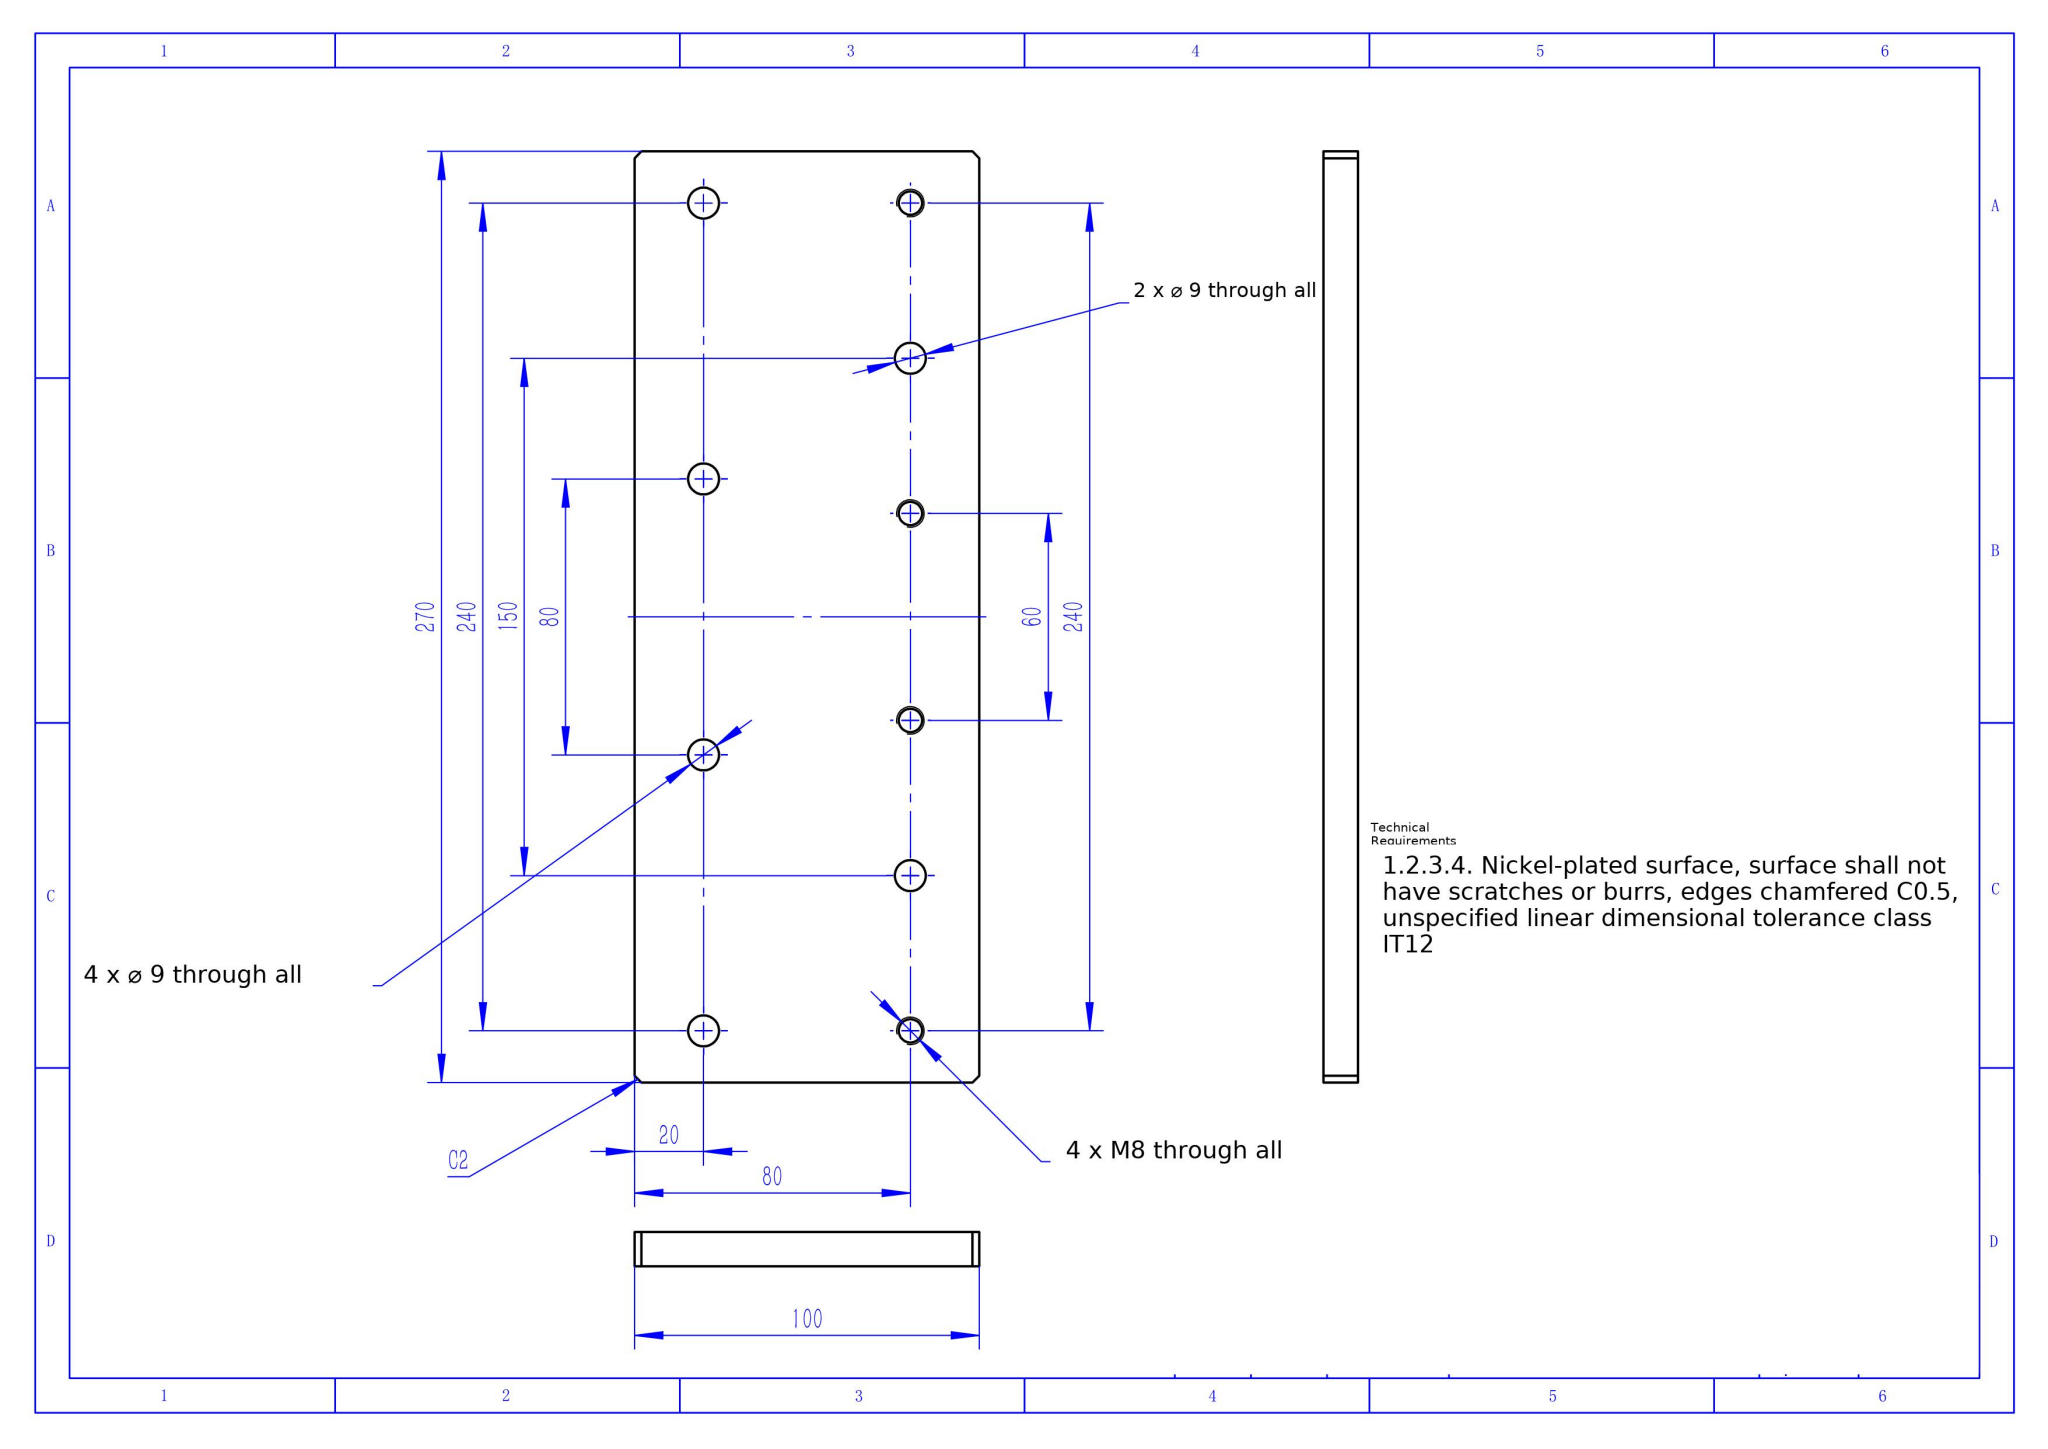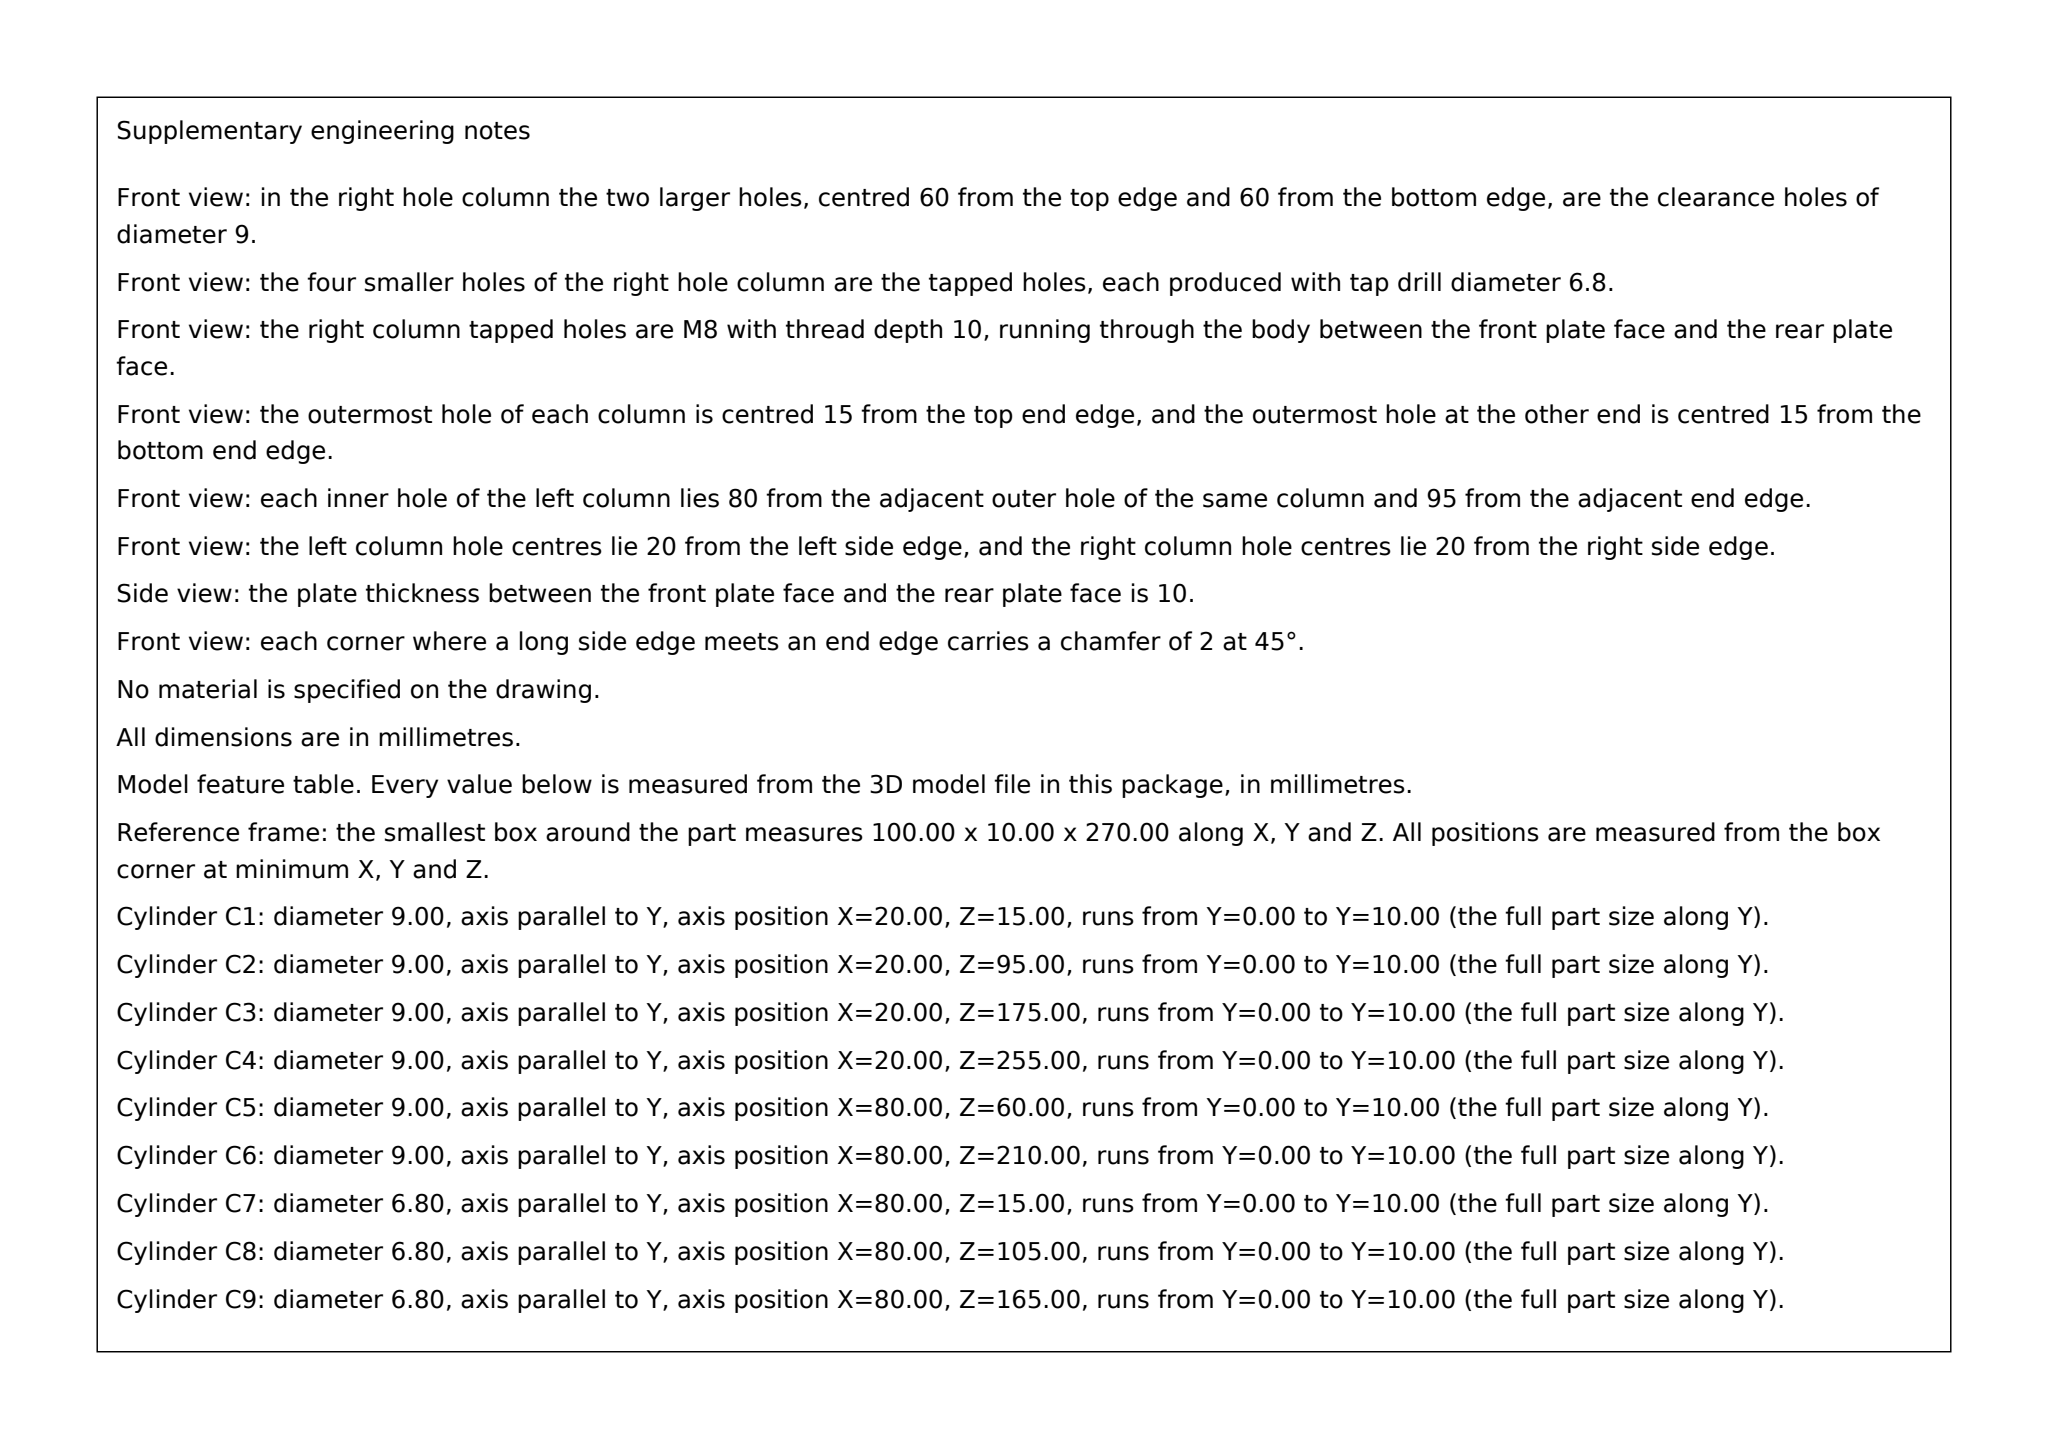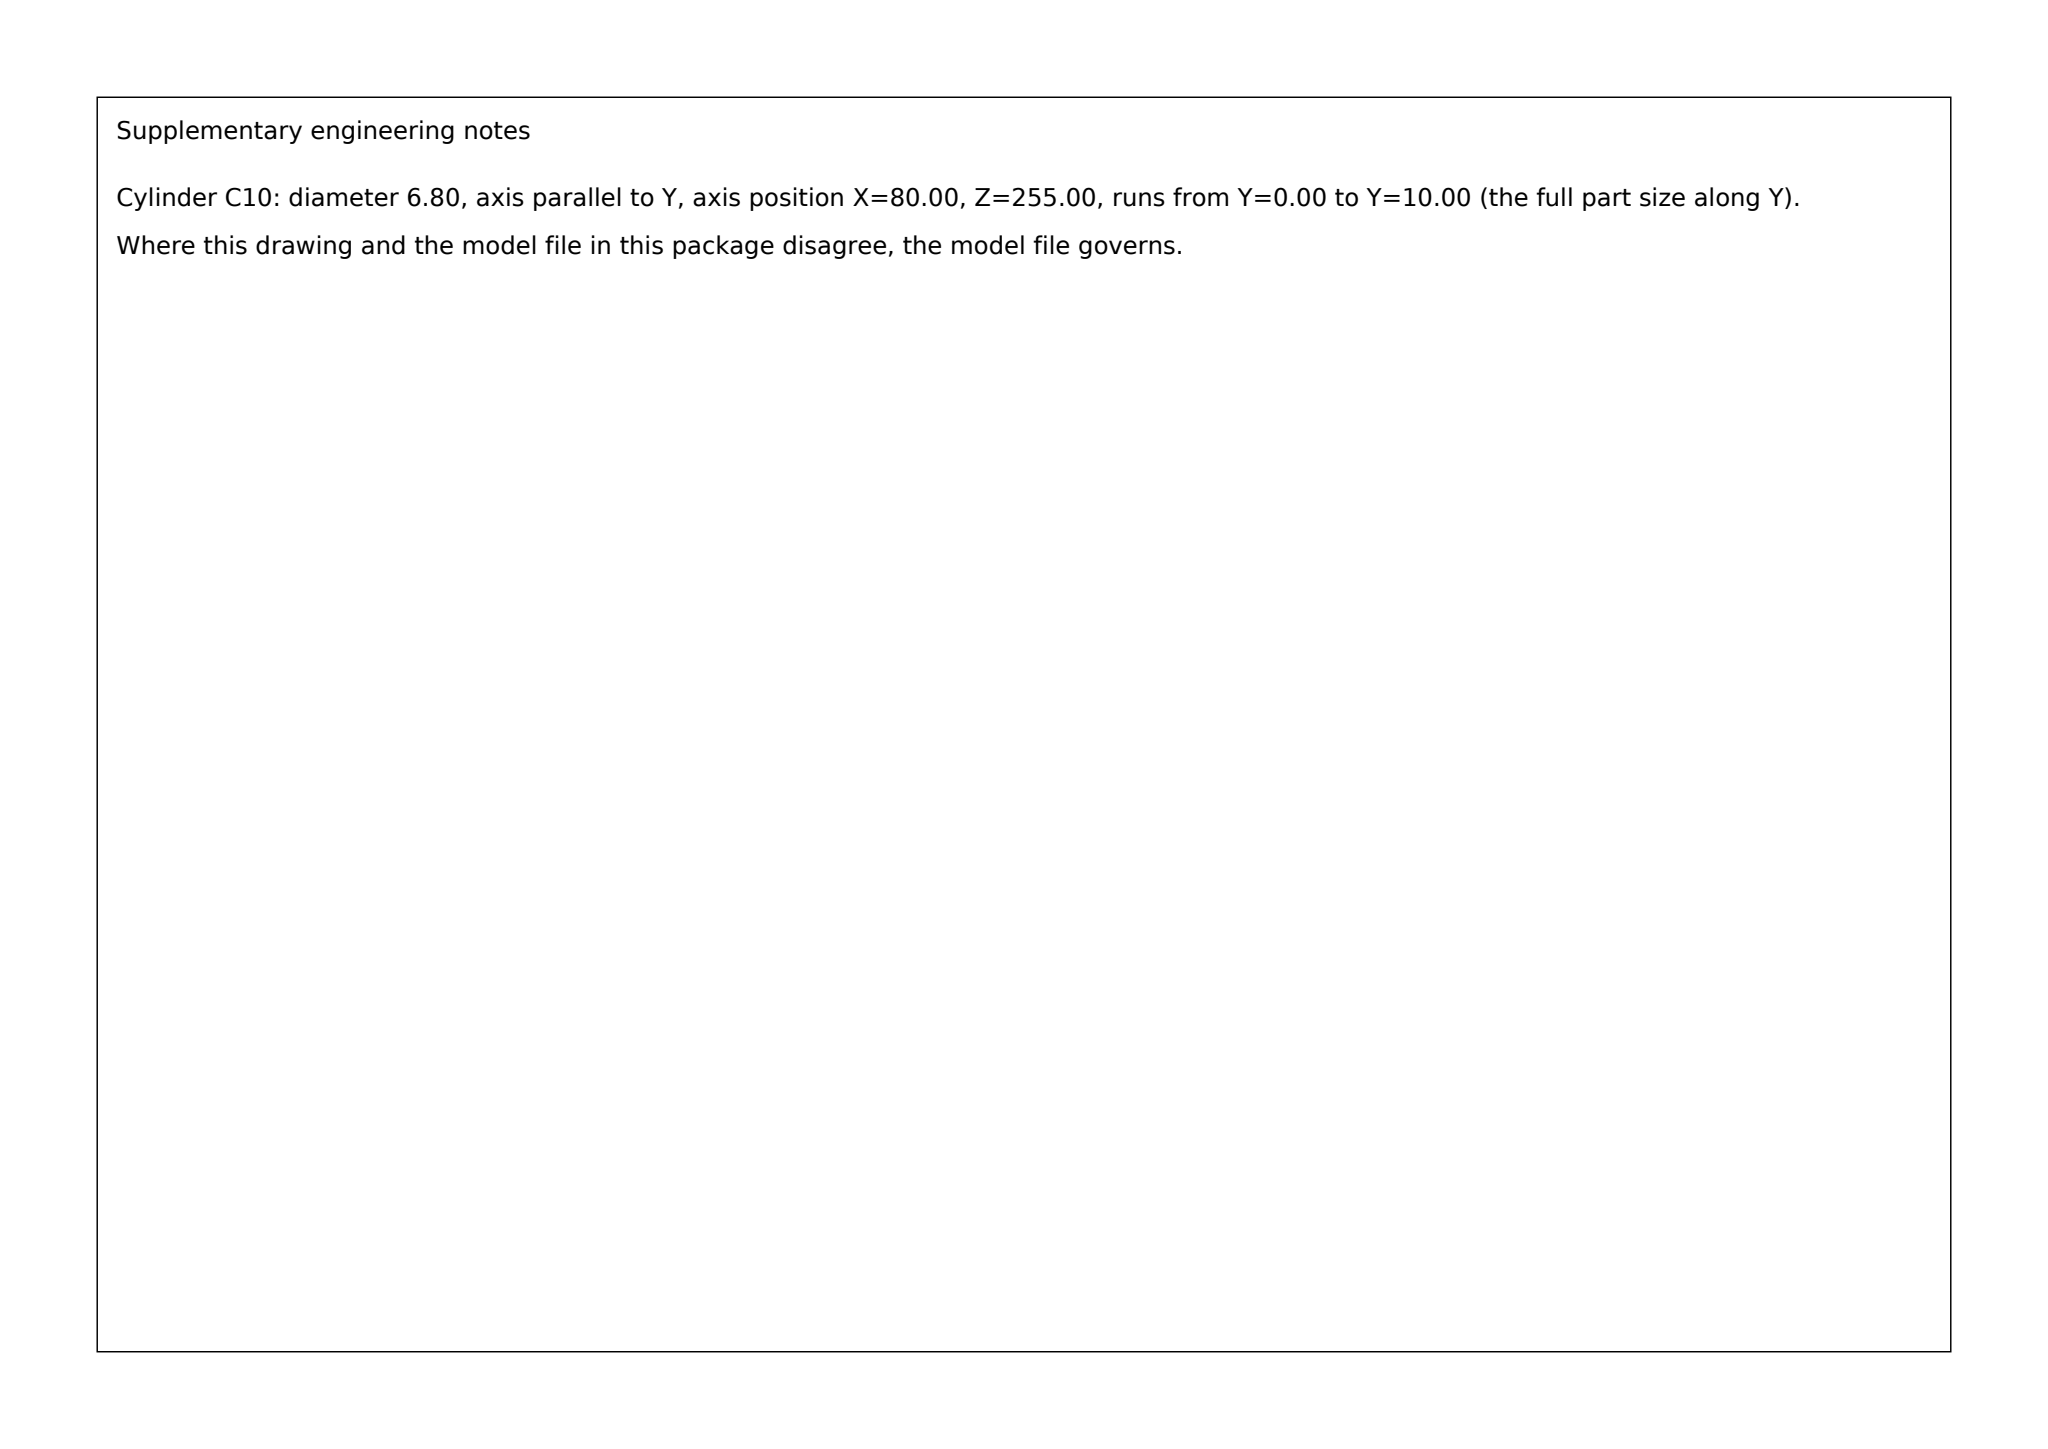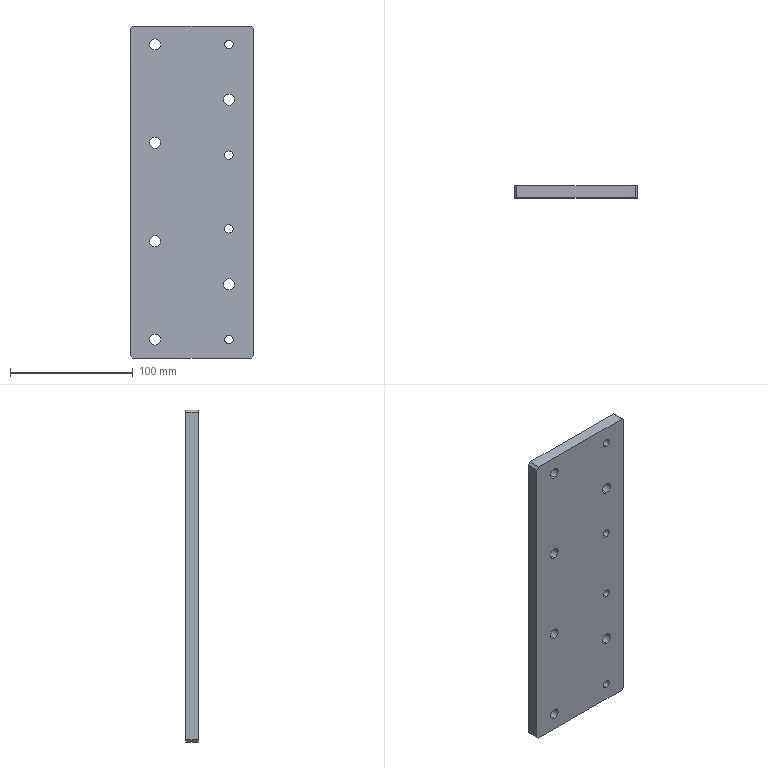Part | SolidWorks | mm | 1 solid | 30 faces | box 100 x 10 x 270 mm | volume 264650 mm3 | cylinder 20 | plane 10 | commonest cylinder face diameters 9 x12 6.8 x8
Drawing notes:
SIDE VIEW: PLATE THK 10 | from the solid: bbox_xyz y = 10.0; y-planes at 0.0 and 10.0; all holes 10 deep
build123d program:
from build123d import *

# Parameters (mm, degrees)
SKETCH1_W            = 100
SKETCH1_H            = 270
BOSS_EXTRUDE1_DEPTH  = 10
M8_CLEARANCE_HOLE1_D = 9
CHAMFER1_SIZE        = 2
M8_CLEARANCE_HOLE2_D = 9
M8_TAPPED_HOLE1_D    = 6.8


with BuildPart() as part:
    # Sketch1 → Boss-Extrude1 (new body)
    with BuildSketch(Plane(origin=(0, 0, 0), x_dir=(1, 0, 0), z_dir=(0, 1, 0))):
        with Locations((30, 0)):
            Rectangle(SKETCH1_W, SKETCH1_H)
    extrude(amount=BOSS_EXTRUDE1_DEPTH)

    # M8 Clearance Hole1 (through all)
    with Locations(Plane(origin=(0, 10, 0), x_dir=(1, 0, 0), z_dir=(0, 1, 0))):
        with Locations((0, 120), (0, 40), (0, -40), (0, -120)):
            Hole(M8_CLEARANCE_HOLE1_D / 2)

    # Chamfer1
    chamfer1_edges = [part.edges().sort_by_distance(p)[0] for p in [
        (-20, 5, -135),
        (80, 5, -135),
        (80, 5, 135),
        (-20, 5, 135),
    ]]
    chamfer(chamfer1_edges, length=CHAMFER1_SIZE)

    # M8 Clearance Hole2 (through all)
    with Locations(Plane(origin=(0, 10, 0), x_dir=(1, 0, 0), z_dir=(0, 1, 0))):
        with Locations((60, 75), (60, -75)):
            Hole(M8_CLEARANCE_HOLE2_D / 2)

    # M8 Tapped Hole1 (through all)
    with Locations(Plane(origin=(0, 10, 0), x_dir=(1, 0, 0), z_dir=(0, 1, 0))):
        with Locations((60, 120), (60, 30), (60, -30), (60, -120)):
            Hole(M8_TAPPED_HOLE1_D / 2)


solid = part.part